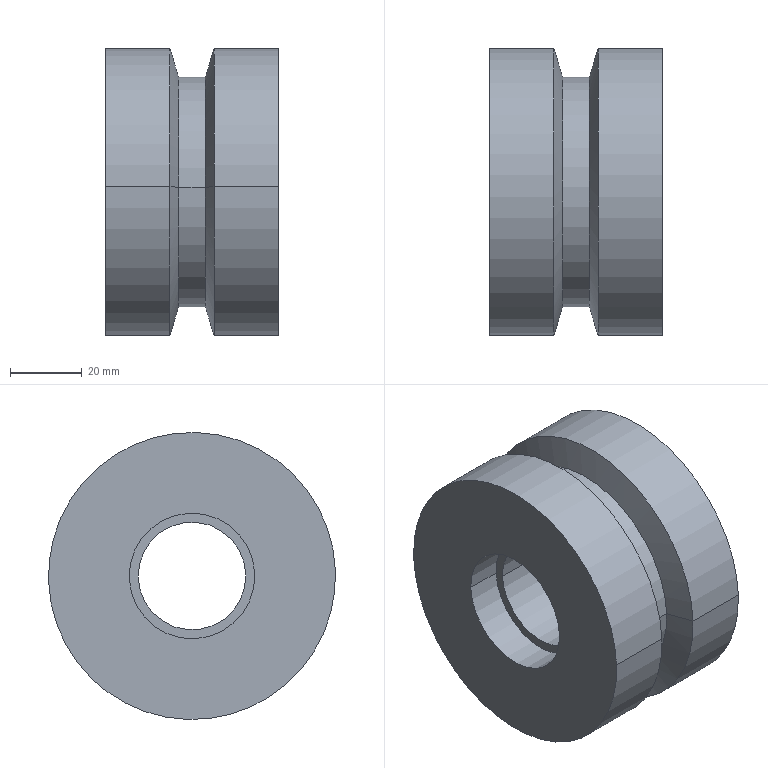Component | SolidWorks | CCD11-00TensioningAssembly-1_CCD05DrivenWheel-1 | 1 solid | 20 faces | box 48 x 80 x 80 mm | volume 184165 mm3 | cylinder 12 | cone 4 | plane 4 | commonest cylinder face diameters 35 x4 80 x4 30 x2 64 x2
build123d program:
from build123d import *


with BuildPart() as part:
    # Sketch1 → Revolve1 (revolve)
    with BuildSketch(Plane.XY, mode=Mode.PRIVATE) as revolve1_sk:
        Polygon((-26.154, 17.5), (-26.154, 40), (-8.304, 40), (-5.904, 32), (1.596, 32), (3.996, 40), (21.846, 40), (21.846, 17.5), (11.846, 17.5), (11.846, 15), (-16.154, 15), (-16.154, 17.5), align=None)
    revolve(revolve1_sk.sketch.rotate(Axis((-155.696, 0, 0), (1, 0, 0)), 90), axis=Axis((-155.696, 0, 0), (1, 0, 0)))


solid = part.part

# Placed as in the assembly
solid = solid.moved(Location((-327.967, 107.251, 149), (0, 0, 0)))
STEP:
#1=COLOUR_RGB('',0.7922,0.8196,0.9333);
#2=FILL_AREA_STYLE_COLOUR('',#1);
#3=FILL_AREA_STYLE('',(#2));
#4=SURFACE_STYLE_FILL_AREA(#3);
#5=SURFACE_SIDE_STYLE('',(#4));
#6=SURFACE_STYLE_USAGE(.BOTH.,#5);
#7=PRESENTATION_STYLE_ASSIGNMENT((#6));
#8=CARTESIAN_POINT('',(-12.446,4.813,5.843));
#9=VERTEX_POINT('',#8);
#10=CARTESIAN_POINT('',(-12.446,3.632,5.889));
#11=VERTEX_POINT('',#10);
#12=CARTESIAN_POINT('',(-12.446,4.222,5.866));
#13=DIRECTION('',(-1.,-0.,0.));
#14=DIRECTION('',(0.,-0.9992,0.03921));
#15=AXIS2_PLACEMENT_3D('',#12,#13,#14);
#16=CIRCLE('',#15,0.5906);
#17=EDGE_CURVE('',#9,#11,#16,.T.);
#18=ORIENTED_EDGE('',*,*,#17,.F.);
#19=CARTESIAN_POINT('',(-13.548,4.813,5.843));
#20=VERTEX_POINT('',#19);
#21=CARTESIAN_POINT('',(-19.042,4.813,5.843));
#22=DIRECTION('',(-1.,-0.,0.));
#23=VECTOR('',#22,39.37);
#24=LINE('',#21,#23);
#25=EDGE_CURVE('',#9,#20,#24,.T.);
#26=ORIENTED_EDGE('',*,*,#25,.T.);
#27=CARTESIAN_POINT('',(-13.548,3.632,5.889));
#28=VERTEX_POINT('',#27);
#29=CARTESIAN_POINT('',(-13.548,4.222,5.866));
#30=DIRECTION('',(-1.,-0.,0.));
#31=DIRECTION('',(0.,-0.9992,0.03921));
#32=AXIS2_PLACEMENT_3D('',#29,#30,#31);
#33=CIRCLE('',#32,0.5906);
#34=EDGE_CURVE('',#20,#28,#33,.T.);
#35=ORIENTED_EDGE('',*,*,#34,.T.);
#36=CARTESIAN_POINT('',(-19.042,3.632,5.889));
#37=DIRECTION('',(-1.,-0.,0.));
#38=VECTOR('',#37,39.37);
#39=LINE('',#36,#38);
#40=EDGE_CURVE('',#11,#28,#39,.T.);
#41=ORIENTED_EDGE('',*,*,#40,.F.);
#42=EDGE_LOOP('',(#18,#26,#35,#41));
#43=FACE_OUTER_BOUND('',#42,.T.);
#44=CARTESIAN_POINT('',(-19.042,4.222,5.866));
#45=DIRECTION('',(-1.,-0.,0.));
#46=DIRECTION('',(0.,-0.9992,0.03921));
#47=AXIS2_PLACEMENT_3D('',#44,#45,#46);
#48=CYLINDRICAL_SURFACE('',#47,0.5906);
#49=ADVANCED_FACE('',(#43),#48,.F.);
#50=CARTESIAN_POINT('',(-12.052,4.911,5.839));
#51=VERTEX_POINT('',#50);
#52=CARTESIAN_POINT('',(-12.052,3.534,5.893));
#53=VERTEX_POINT('',#52);
#54=CARTESIAN_POINT('',(-12.052,4.222,5.866));
#55=DIRECTION('',(-1.,-0.,0.));
#56=DIRECTION('',(0.,-0.9992,0.03921));
#57=AXIS2_PLACEMENT_3D('',#54,#55,#56);
#58=CIRCLE('',#57,0.689);
#59=EDGE_CURVE('',#51,#53,#58,.T.);
#60=ORIENTED_EDGE('',*,*,#59,.F.);
#61=CARTESIAN_POINT('',(-12.446,4.911,5.839));
#62=VERTEX_POINT('',#61);
#63=CARTESIAN_POINT('',(-19.042,4.911,5.839));
#64=DIRECTION('',(-1.,-0.,0.));
#65=VECTOR('',#64,39.37);
#66=LINE('',#63,#65);
#67=EDGE_CURVE('',#51,#62,#66,.T.);
#68=ORIENTED_EDGE('',*,*,#67,.T.);
#69=CARTESIAN_POINT('',(-12.446,3.534,5.893));
#70=VERTEX_POINT('',#69);
#71=CARTESIAN_POINT('',(-12.446,4.222,5.866));
#72=DIRECTION('',(-1.,-0.,0.));
#73=DIRECTION('',(0.,-0.9992,0.03921));
#74=AXIS2_PLACEMENT_3D('',#71,#72,#73);
#75=CIRCLE('',#74,0.689);
#76=EDGE_CURVE('',#62,#70,#75,.T.);
#77=ORIENTED_EDGE('',*,*,#76,.T.);
#78=CARTESIAN_POINT('',(-19.042,3.534,5.893));
#79=DIRECTION('',(-1.,-0.,0.));
#80=VECTOR('',#79,39.37);
#81=LINE('',#78,#80);
#82=EDGE_CURVE('',#53,#70,#81,.T.);
#83=ORIENTED_EDGE('',*,*,#82,.F.);
#84=EDGE_LOOP('',(#60,#68,#77,#83));
#85=FACE_OUTER_BOUND('',#84,.T.);
#86=CARTESIAN_POINT('',(-19.042,4.222,5.866));
#87=DIRECTION('',(-1.,-0.,0.));
#88=DIRECTION('',(0.,-0.9992,0.03921));
#89=AXIS2_PLACEMENT_3D('',#86,#87,#88);
#90=CYLINDRICAL_SURFACE('',#89,0.689);
#91=ADVANCED_FACE('',(#85),#90,.F.);
#92=CARTESIAN_POINT('',(-12.052,2.649,5.928));
#93=VERTEX_POINT('',#92);
#94=CARTESIAN_POINT('',(-12.052,5.796,5.804));
#95=VERTEX_POINT('',#94);
#96=CARTESIAN_POINT('',(-12.052,4.222,5.866));
#97=DIRECTION('',(-1.,-0.,0.));
#98=DIRECTION('',(0.,-0.9992,0.03921));
#99=AXIS2_PLACEMENT_3D('',#96,#97,#98);
#100=CIRCLE('',#99,1.575);
#101=EDGE_CURVE('',#93,#95,#100,.T.);
#102=ORIENTED_EDGE('',*,*,#101,.T.);
#103=CARTESIAN_POINT('',(-12.755,5.796,5.804));
#104=VERTEX_POINT('',#103);
#105=CARTESIAN_POINT('',(-19.042,5.796,5.804));
#106=DIRECTION('',(-1.,-0.,0.));
#107=VECTOR('',#106,39.37);
#108=LINE('',#105,#107);
#109=EDGE_CURVE('',#95,#104,#108,.T.);
#110=ORIENTED_EDGE('',*,*,#109,.T.);
#111=CARTESIAN_POINT('',(-12.755,2.649,5.928));
#112=VERTEX_POINT('',#111);
#113=CARTESIAN_POINT('',(-12.755,4.222,5.866));
#114=DIRECTION('',(-1.,-0.,0.));
#115=DIRECTION('',(0.,-0.9992,0.03921));
#116=AXIS2_PLACEMENT_3D('',#113,#114,#115);
#117=CIRCLE('',#116,1.575);
#118=EDGE_CURVE('',#112,#104,#117,.T.);
#119=ORIENTED_EDGE('',*,*,#118,.F.);
#120=CARTESIAN_POINT('',(-19.042,2.649,5.928));
#121=DIRECTION('',(-1.,-0.,0.));
#122=VECTOR('',#121,39.37);
#123=LINE('',#120,#122);
#124=EDGE_CURVE('',#93,#112,#123,.T.);
#125=ORIENTED_EDGE('',*,*,#124,.F.);
#126=EDGE_LOOP('',(#102,#110,#119,#125));
#127=FACE_OUTER_BOUND('',#126,.T.);
#128=CARTESIAN_POINT('',(-19.042,4.222,5.866));
#129=DIRECTION('',(-1.,-0.,0.));
#130=DIRECTION('',(0.,-0.9992,0.03921));
#131=AXIS2_PLACEMENT_3D('',#128,#129,#130);
#132=CYLINDRICAL_SURFACE('',#131,1.575);
#133=ADVANCED_FACE('',(#127),#132,.T.);
#134=CARTESIAN_POINT('',(-12.849,2.964,5.916));
#135=VERTEX_POINT('',#134);
#136=CARTESIAN_POINT('',(-12.849,5.481,5.817));
#137=VERTEX_POINT('',#136);
#138=CARTESIAN_POINT('',(-12.849,4.222,5.866));
#139=DIRECTION('',(-1.,-0.,0.));
#140=DIRECTION('',(0.,-0.9992,0.03921));
#141=AXIS2_PLACEMENT_3D('',#138,#139,#140);
#142=CIRCLE('',#141,1.26);
#143=EDGE_CURVE('',#135,#137,#142,.T.);
#144=ORIENTED_EDGE('',*,*,#143,.F.);
#145=CARTESIAN_POINT('',(-12.755,2.649,5.928));
#146=DIRECTION('',(0.2873,-0.9571,0.03756));
#147=VECTOR('',#146,39.37);
#148=LINE('',#145,#147);
#149=EDGE_CURVE('',#135,#112,#148,.T.);
#150=ORIENTED_EDGE('',*,*,#149,.T.);
#151=ORIENTED_EDGE('',*,*,#118,.T.);
#152=CARTESIAN_POINT('',(-12.755,5.796,5.804));
#153=DIRECTION('',(0.2873,0.9571,-0.03756));
#154=VECTOR('',#153,39.37);
#155=LINE('',#152,#154);
#156=EDGE_CURVE('',#137,#104,#155,.T.);
#157=ORIENTED_EDGE('',*,*,#156,.F.);
#158=EDGE_LOOP('',(#144,#150,#151,#157));
#159=FACE_OUTER_BOUND('',#158,.T.);
#160=CARTESIAN_POINT('',(-12.755,4.222,5.866));
#161=DIRECTION('',(1.,0.,-0.));
#162=DIRECTION('',(-0.,0.9992,-0.03921));
#163=AXIS2_PLACEMENT_3D('',#160,#161,#162);
#164=CONICAL_SURFACE('',#163,1.575,1.279);
#165=ADVANCED_FACE('',(#159),#164,.T.);
#166=ORIENTED_EDGE('',*,*,#143,.T.);
#167=CARTESIAN_POINT('',(-13.145,5.481,5.817));
#168=VERTEX_POINT('',#167);
#169=CARTESIAN_POINT('',(-19.042,5.481,5.817));
#170=DIRECTION('',(-1.,-0.,0.));
#171=VECTOR('',#170,39.37);
#172=LINE('',#169,#171);
#173=EDGE_CURVE('',#137,#168,#172,.T.);
#174=ORIENTED_EDGE('',*,*,#173,.T.);
#175=CARTESIAN_POINT('',(-13.145,2.964,5.916));
#176=VERTEX_POINT('',#175);
#177=CARTESIAN_POINT('',(-13.145,4.222,5.866));
#178=DIRECTION('',(-1.,-0.,0.));
#179=DIRECTION('',(0.,-0.9992,0.03921));
#180=AXIS2_PLACEMENT_3D('',#177,#178,#179);
#181=CIRCLE('',#180,1.26);
#182=EDGE_CURVE('',#176,#168,#181,.T.);
#183=ORIENTED_EDGE('',*,*,#182,.F.);
#184=CARTESIAN_POINT('',(-19.042,2.964,5.916));
#185=DIRECTION('',(-1.,-0.,0.));
#186=VECTOR('',#185,39.37);
#187=LINE('',#184,#186);
#188=EDGE_CURVE('',#135,#176,#187,.T.);
#189=ORIENTED_EDGE('',*,*,#188,.F.);
#190=EDGE_LOOP('',(#166,#174,#183,#189));
#191=FACE_OUTER_BOUND('',#190,.T.);
#192=CARTESIAN_POINT('',(-19.042,4.222,5.866));
#193=DIRECTION('',(-1.,-0.,0.));
#194=DIRECTION('',(0.,-0.9992,0.03921));
#195=AXIS2_PLACEMENT_3D('',#192,#193,#194);
#196=CYLINDRICAL_SURFACE('',#195,1.26);
#197=ADVANCED_FACE('',(#191),#196,.T.);
#198=ORIENTED_EDGE('',*,*,#182,.T.);
#199=CARTESIAN_POINT('',(-13.239,5.796,5.804));
#200=VERTEX_POINT('',#199);
#201=CARTESIAN_POINT('',(-13.145,5.481,5.817));
#202=DIRECTION('',(-0.2873,0.9571,-0.03756));
#203=VECTOR('',#202,39.37);
#204=LINE('',#201,#203);
#205=EDGE_CURVE('',#168,#200,#204,.T.);
#206=ORIENTED_EDGE('',*,*,#205,.T.);
#207=CARTESIAN_POINT('',(-13.239,2.649,5.928));
#208=VERTEX_POINT('',#207);
#209=CARTESIAN_POINT('',(-13.239,4.222,5.866));
#210=DIRECTION('',(-1.,-0.,0.));
#211=DIRECTION('',(0.,-0.9992,0.03921));
#212=AXIS2_PLACEMENT_3D('',#209,#210,#211);
#213=CIRCLE('',#212,1.575);
#214=EDGE_CURVE('',#208,#200,#213,.T.);
#215=ORIENTED_EDGE('',*,*,#214,.F.);
#216=CARTESIAN_POINT('',(-13.145,2.964,5.916));
#217=DIRECTION('',(-0.2873,-0.9571,0.03756));
#218=VECTOR('',#217,39.37);
#219=LINE('',#216,#218);
#220=EDGE_CURVE('',#176,#208,#219,.T.);
#221=ORIENTED_EDGE('',*,*,#220,.F.);
#222=EDGE_LOOP('',(#198,#206,#215,#221));
#223=FACE_OUTER_BOUND('',#222,.T.);
#224=CARTESIAN_POINT('',(-13.145,4.222,5.866));
#225=DIRECTION('',(-1.,-0.,0.));
#226=DIRECTION('',(0.,-0.9992,0.03921));
#227=AXIS2_PLACEMENT_3D('',#224,#225,#226);
#228=CONICAL_SURFACE('',#227,1.26,1.279);
#229=ADVANCED_FACE('',(#223),#228,.T.);
#230=ORIENTED_EDGE('',*,*,#214,.T.);
#231=CARTESIAN_POINT('',(-13.942,5.796,5.804));
#232=VERTEX_POINT('',#231);
#233=CARTESIAN_POINT('',(-19.042,5.796,5.804));
#234=DIRECTION('',(-1.,-0.,0.));
#235=VECTOR('',#234,39.37);
#236=LINE('',#233,#235);
#237=EDGE_CURVE('',#200,#232,#236,.T.);
#238=ORIENTED_EDGE('',*,*,#237,.T.);
#239=CARTESIAN_POINT('',(-13.942,2.649,5.928));
#240=VERTEX_POINT('',#239);
#241=CARTESIAN_POINT('',(-13.942,4.222,5.866));
#242=DIRECTION('',(-1.,-0.,0.));
#243=DIRECTION('',(0.,-0.9992,0.03921));
#244=AXIS2_PLACEMENT_3D('',#241,#242,#243);
#245=CIRCLE('',#244,1.575);
#246=EDGE_CURVE('',#240,#232,#245,.T.);
#247=ORIENTED_EDGE('',*,*,#246,.F.);
#248=CARTESIAN_POINT('',(-19.042,2.649,5.928));
#249=DIRECTION('',(-1.,-0.,0.));
#250=VECTOR('',#249,39.37);
#251=LINE('',#248,#250);
#252=EDGE_CURVE('',#208,#240,#251,.T.);
#253=ORIENTED_EDGE('',*,*,#252,.F.);
#254=EDGE_LOOP('',(#230,#238,#247,#253));
#255=FACE_OUTER_BOUND('',#254,.T.);
#256=CARTESIAN_POINT('',(-19.042,4.222,5.866));
#257=DIRECTION('',(-1.,-0.,0.));
#258=DIRECTION('',(0.,-0.9992,0.03921));
#259=AXIS2_PLACEMENT_3D('',#256,#257,#258);
#260=CYLINDRICAL_SURFACE('',#259,1.575);
#261=ADVANCED_FACE('',(#255),#260,.T.);
#262=CARTESIAN_POINT('',(-13.548,4.911,5.839));
#263=VERTEX_POINT('',#262);
#264=CARTESIAN_POINT('',(-13.548,3.534,5.893));
#265=VERTEX_POINT('',#264);
#266=CARTESIAN_POINT('',(-13.548,4.222,5.866));
#267=DIRECTION('',(-1.,-0.,0.));
#268=DIRECTION('',(0.,-0.9992,0.03921));
#269=AXIS2_PLACEMENT_3D('',#266,#267,#268);
#270=CIRCLE('',#269,0.689);
#271=EDGE_CURVE('',#263,#265,#270,.T.);
#272=ORIENTED_EDGE('',*,*,#271,.F.);
#273=CARTESIAN_POINT('',(-13.942,4.911,5.839));
#274=VERTEX_POINT('',#273);
#275=CARTESIAN_POINT('',(-19.042,4.911,5.839));
#276=DIRECTION('',(-1.,-0.,0.));
#277=VECTOR('',#276,39.37);
#278=LINE('',#275,#277);
#279=EDGE_CURVE('',#263,#274,#278,.T.);
#280=ORIENTED_EDGE('',*,*,#279,.T.);
#281=CARTESIAN_POINT('',(-13.942,3.534,5.893));
#282=VERTEX_POINT('',#281);
#283=CARTESIAN_POINT('',(-13.942,4.222,5.866));
#284=DIRECTION('',(-1.,-0.,0.));
#285=DIRECTION('',(0.,-0.9992,0.03921));
#286=AXIS2_PLACEMENT_3D('',#283,#284,#285);
#287=CIRCLE('',#286,0.689);
#288=EDGE_CURVE('',#274,#282,#287,.T.);
#289=ORIENTED_EDGE('',*,*,#288,.T.);
#290=CARTESIAN_POINT('',(-19.042,3.534,5.893));
#291=DIRECTION('',(-1.,-0.,0.));
#292=VECTOR('',#291,39.37);
#293=LINE('',#290,#292);
#294=EDGE_CURVE('',#265,#282,#293,.T.);
#295=ORIENTED_EDGE('',*,*,#294,.F.);
#296=EDGE_LOOP('',(#272,#280,#289,#295));
#297=FACE_OUTER_BOUND('',#296,.T.);
#298=CARTESIAN_POINT('',(-19.042,4.222,5.866));
#299=DIRECTION('',(-1.,-0.,0.));
#300=DIRECTION('',(0.,-0.9992,0.03921));
#301=AXIS2_PLACEMENT_3D('',#298,#299,#300);
#302=CYLINDRICAL_SURFACE('',#301,0.689);
#303=ADVANCED_FACE('',(#297),#302,.F.);
#304=ORIENTED_EDGE('',*,*,#279,.F.);
#305=CARTESIAN_POINT('',(-13.548,4.222,5.866));
#306=DIRECTION('',(-1.,-0.,0.));
#307=DIRECTION('',(0.,-0.9992,0.03921));
#308=AXIS2_PLACEMENT_3D('',#305,#306,#307);
#309=CIRCLE('',#308,0.689);
#310=EDGE_CURVE('',#265,#263,#309,.T.);
#311=ORIENTED_EDGE('',*,*,#310,.F.);
#312=ORIENTED_EDGE('',*,*,#294,.T.);
#313=CARTESIAN_POINT('',(-13.942,4.222,5.866));
#314=DIRECTION('',(-1.,-0.,0.));
#315=DIRECTION('',(0.,-0.9992,0.03921));
#316=AXIS2_PLACEMENT_3D('',#313,#314,#315);
#317=CIRCLE('',#316,0.689);
#318=EDGE_CURVE('',#282,#274,#317,.T.);
#319=ORIENTED_EDGE('',*,*,#318,.T.);
#320=EDGE_LOOP('',(#304,#311,#312,#319));
#321=FACE_OUTER_BOUND('',#320,.T.);
#322=CARTESIAN_POINT('',(-19.042,4.222,5.866));
#323=DIRECTION('',(-1.,-0.,0.));
#324=DIRECTION('',(0.,-0.9992,0.03921));
#325=AXIS2_PLACEMENT_3D('',#322,#323,#324);
#326=CYLINDRICAL_SURFACE('',#325,0.689);
#327=ADVANCED_FACE('',(#321),#326,.F.);
#328=ORIENTED_EDGE('',*,*,#318,.F.);
#329=ORIENTED_EDGE('',*,*,#288,.F.);
#330=EDGE_LOOP('',(#328,#329));
#331=FACE_BOUND('',#330,.T.);
#332=ORIENTED_EDGE('',*,*,#246,.T.);
#333=CARTESIAN_POINT('',(-13.942,4.222,5.866));
#334=DIRECTION('',(-1.,-0.,0.));
#335=DIRECTION('',(0.,-0.9992,0.03921));
#336=AXIS2_PLACEMENT_3D('',#333,#334,#335);
#337=CIRCLE('',#336,1.575);
#338=EDGE_CURVE('',#232,#240,#337,.T.);
#339=ORIENTED_EDGE('',*,*,#338,.T.);
#340=EDGE_LOOP('',(#332,#339));
#341=FACE_OUTER_BOUND('',#340,.T.);
#342=CARTESIAN_POINT('',(-13.942,4.25,6.555));
#343=DIRECTION('',(1.,0.,-0.));
#344=DIRECTION('',(-0.,0.9992,-0.03921));
#345=AXIS2_PLACEMENT_3D('',#342,#343,#344);
#346=PLANE('',#345);
#347=ADVANCED_FACE('',(#331,#341),#346,.F.);
#348=ORIENTED_EDGE('',*,*,#237,.F.);
#349=CARTESIAN_POINT('',(-13.239,4.222,5.866));
#350=DIRECTION('',(-1.,-0.,0.));
#351=DIRECTION('',(0.,-0.9992,0.03921));
#352=AXIS2_PLACEMENT_3D('',#349,#350,#351);
#353=CIRCLE('',#352,1.575);
#354=EDGE_CURVE('',#200,#208,#353,.T.);
#355=ORIENTED_EDGE('',*,*,#354,.T.);
#356=ORIENTED_EDGE('',*,*,#252,.T.);
#357=ORIENTED_EDGE('',*,*,#338,.F.);
#358=EDGE_LOOP('',(#348,#355,#356,#357));
#359=FACE_OUTER_BOUND('',#358,.T.);
#360=CARTESIAN_POINT('',(-19.042,4.222,5.866));
#361=DIRECTION('',(-1.,-0.,0.));
#362=DIRECTION('',(0.,-0.9992,0.03921));
#363=AXIS2_PLACEMENT_3D('',#360,#361,#362);
#364=CYLINDRICAL_SURFACE('',#363,1.575);
#365=ADVANCED_FACE('',(#359),#364,.T.);
#366=ORIENTED_EDGE('',*,*,#205,.F.);
#367=CARTESIAN_POINT('',(-13.145,4.222,5.866));
#368=DIRECTION('',(-1.,-0.,0.));
#369=DIRECTION('',(0.,-0.9992,0.03921));
#370=AXIS2_PLACEMENT_3D('',#367,#368,#369);
#371=CIRCLE('',#370,1.26);
#372=EDGE_CURVE('',#168,#176,#371,.T.);
#373=ORIENTED_EDGE('',*,*,#372,.T.);
#374=ORIENTED_EDGE('',*,*,#220,.T.);
#375=ORIENTED_EDGE('',*,*,#354,.F.);
#376=EDGE_LOOP('',(#366,#373,#374,#375));
#377=FACE_OUTER_BOUND('',#376,.T.);
#378=CARTESIAN_POINT('',(-13.145,4.222,5.866));
#379=DIRECTION('',(-1.,-0.,0.));
#380=DIRECTION('',(0.,-0.9992,0.03921));
#381=AXIS2_PLACEMENT_3D('',#378,#379,#380);
#382=CONICAL_SURFACE('',#381,1.26,1.279);
#383=ADVANCED_FACE('',(#377),#382,.T.);
#384=ORIENTED_EDGE('',*,*,#173,.F.);
#385=CARTESIAN_POINT('',(-12.849,4.222,5.866));
#386=DIRECTION('',(-1.,-0.,0.));
#387=DIRECTION('',(0.,-0.9992,0.03921));
#388=AXIS2_PLACEMENT_3D('',#385,#386,#387);
#389=CIRCLE('',#388,1.26);
#390=EDGE_CURVE('',#137,#135,#389,.T.);
#391=ORIENTED_EDGE('',*,*,#390,.T.);
#392=ORIENTED_EDGE('',*,*,#188,.T.);
#393=ORIENTED_EDGE('',*,*,#372,.F.);
#394=EDGE_LOOP('',(#384,#391,#392,#393));
#395=FACE_OUTER_BOUND('',#394,.T.);
#396=CARTESIAN_POINT('',(-19.042,4.222,5.866));
#397=DIRECTION('',(-1.,-0.,0.));
#398=DIRECTION('',(0.,-0.9992,0.03921));
#399=AXIS2_PLACEMENT_3D('',#396,#397,#398);
#400=CYLINDRICAL_SURFACE('',#399,1.26);
#401=ADVANCED_FACE('',(#395),#400,.T.);
#402=ORIENTED_EDGE('',*,*,#149,.F.);
#403=ORIENTED_EDGE('',*,*,#390,.F.);
#404=ORIENTED_EDGE('',*,*,#156,.T.);
#405=CARTESIAN_POINT('',(-12.755,4.222,5.866));
#406=DIRECTION('',(-1.,-0.,0.));
#407=DIRECTION('',(0.,-0.9992,0.03921));
#408=AXIS2_PLACEMENT_3D('',#405,#406,#407);
#409=CIRCLE('',#408,1.575);
#410=EDGE_CURVE('',#104,#112,#409,.T.);
#411=ORIENTED_EDGE('',*,*,#410,.T.);
#412=EDGE_LOOP('',(#402,#403,#404,#411));
#413=FACE_OUTER_BOUND('',#412,.T.);
#414=CARTESIAN_POINT('',(-12.755,4.222,5.866));
#415=DIRECTION('',(1.,0.,-0.));
#416=DIRECTION('',(-0.,0.9992,-0.03921));
#417=AXIS2_PLACEMENT_3D('',#414,#415,#416);
#418=CONICAL_SURFACE('',#417,1.575,1.279);
#419=ADVANCED_FACE('',(#413),#418,.T.);
#420=ORIENTED_EDGE('',*,*,#109,.F.);
#421=CARTESIAN_POINT('',(-12.052,4.222,5.866));
#422=DIRECTION('',(-1.,-0.,0.));
#423=DIRECTION('',(0.,-0.9992,0.03921));
#424=AXIS2_PLACEMENT_3D('',#421,#422,#423);
#425=CIRCLE('',#424,1.575);
#426=EDGE_CURVE('',#95,#93,#425,.T.);
#427=ORIENTED_EDGE('',*,*,#426,.T.);
#428=ORIENTED_EDGE('',*,*,#124,.T.);
#429=ORIENTED_EDGE('',*,*,#410,.F.);
#430=EDGE_LOOP('',(#420,#427,#428,#429));
#431=FACE_OUTER_BOUND('',#430,.T.);
#432=CARTESIAN_POINT('',(-19.042,4.222,5.866));
#433=DIRECTION('',(-1.,-0.,0.));
#434=DIRECTION('',(0.,-0.9992,0.03921));
#435=AXIS2_PLACEMENT_3D('',#432,#433,#434);
#436=CYLINDRICAL_SURFACE('',#435,1.575);
#437=ADVANCED_FACE('',(#431),#436,.T.);
#438=ORIENTED_EDGE('',*,*,#101,.F.);
#439=ORIENTED_EDGE('',*,*,#426,.F.);
#440=EDGE_LOOP('',(#438,#439));
#441=FACE_OUTER_BOUND('',#440,.T.);
#442=CARTESIAN_POINT('',(-12.052,4.222,5.866));
#443=DIRECTION('',(-1.,-0.,0.));
#444=DIRECTION('',(0.,-0.9992,0.03921));
#445=AXIS2_PLACEMENT_3D('',#442,#443,#444);
#446=CIRCLE('',#445,0.689);
#447=EDGE_CURVE('',#53,#51,#446,.T.);
#448=ORIENTED_EDGE('',*,*,#447,.T.);
#449=ORIENTED_EDGE('',*,*,#59,.T.);
#450=EDGE_LOOP('',(#448,#449));
#451=FACE_BOUND('',#450,.T.);
#452=CARTESIAN_POINT('',(-12.052,4.284,7.44));
#453=DIRECTION('',(-1.,-0.,0.));
#454=DIRECTION('',(0.,-0.9992,0.03921));
#455=AXIS2_PLACEMENT_3D('',#452,#453,#454);
#456=PLANE('',#455);
#457=ADVANCED_FACE('',(#441,#451),#456,.F.);
#458=ORIENTED_EDGE('',*,*,#67,.F.);
#459=ORIENTED_EDGE('',*,*,#447,.F.);
#460=ORIENTED_EDGE('',*,*,#82,.T.);
#461=CARTESIAN_POINT('',(-12.446,4.222,5.866));
#462=DIRECTION('',(-1.,-0.,0.));
#463=DIRECTION('',(0.,-0.9992,0.03921));
#464=AXIS2_PLACEMENT_3D('',#461,#462,#463);
#465=CIRCLE('',#464,0.689);
#466=EDGE_CURVE('',#70,#62,#465,.T.);
#467=ORIENTED_EDGE('',*,*,#466,.T.);
#468=EDGE_LOOP('',(#458,#459,#460,#467));
#469=FACE_OUTER_BOUND('',#468,.T.);
#470=CARTESIAN_POINT('',(-19.042,4.222,5.866));
#471=DIRECTION('',(-1.,-0.,0.));
#472=DIRECTION('',(0.,-0.9992,0.03921));
#473=AXIS2_PLACEMENT_3D('',#470,#471,#472);
#474=CYLINDRICAL_SURFACE('',#473,0.689);
#475=ADVANCED_FACE('',(#469),#474,.F.);
#476=ORIENTED_EDGE('',*,*,#466,.F.);
#477=ORIENTED_EDGE('',*,*,#76,.F.);
#478=EDGE_LOOP('',(#476,#477));
#479=FACE_OUTER_BOUND('',#478,.T.);
#480=CARTESIAN_POINT('',(-12.446,4.222,5.866));
#481=DIRECTION('',(-1.,-0.,0.));
#482=DIRECTION('',(0.,-0.9992,0.03921));
#483=AXIS2_PLACEMENT_3D('',#480,#481,#482);
#484=CIRCLE('',#483,0.5906);
#485=EDGE_CURVE('',#11,#9,#484,.T.);
#486=ORIENTED_EDGE('',*,*,#485,.T.);
#487=ORIENTED_EDGE('',*,*,#17,.T.);
#488=EDGE_LOOP('',(#486,#487));
#489=FACE_BOUND('',#488,.T.);
#490=CARTESIAN_POINT('',(-12.446,4.25,6.555));
#491=DIRECTION('',(-1.,-0.,0.));
#492=DIRECTION('',(0.,-0.9992,0.03921));
#493=AXIS2_PLACEMENT_3D('',#490,#491,#492);
#494=PLANE('',#493);
#495=ADVANCED_FACE('',(#479,#489),#494,.F.);
#496=ORIENTED_EDGE('',*,*,#25,.F.);
#497=ORIENTED_EDGE('',*,*,#485,.F.);
#498=ORIENTED_EDGE('',*,*,#40,.T.);
#499=CARTESIAN_POINT('',(-13.548,4.222,5.866));
#500=DIRECTION('',(-1.,-0.,0.));
#501=DIRECTION('',(0.,-0.9992,0.03921));
#502=AXIS2_PLACEMENT_3D('',#499,#500,#501);
#503=CIRCLE('',#502,0.5906);
#504=EDGE_CURVE('',#28,#20,#503,.T.);
#505=ORIENTED_EDGE('',*,*,#504,.T.);
#506=EDGE_LOOP('',(#496,#497,#498,#505));
#507=FACE_OUTER_BOUND('',#506,.T.);
#508=CARTESIAN_POINT('',(-19.042,4.222,5.866));
#509=DIRECTION('',(-1.,-0.,0.));
#510=DIRECTION('',(0.,-0.9992,0.03921));
#511=AXIS2_PLACEMENT_3D('',#508,#509,#510);
#512=CYLINDRICAL_SURFACE('',#511,0.5906);
#513=ADVANCED_FACE('',(#507),#512,.F.);
#514=ORIENTED_EDGE('',*,*,#504,.F.);
#515=ORIENTED_EDGE('',*,*,#34,.F.);
#516=EDGE_LOOP('',(#514,#515));
#517=FACE_BOUND('',#516,.T.);
#518=ORIENTED_EDGE('',*,*,#310,.T.);
#519=ORIENTED_EDGE('',*,*,#271,.T.);
#520=EDGE_LOOP('',(#518,#519));
#521=FACE_OUTER_BOUND('',#520,.T.);
#522=CARTESIAN_POINT('',(-13.548,4.246,6.456));
#523=DIRECTION('',(1.,0.,-0.));
#524=DIRECTION('',(-0.,0.9992,-0.03921));
#525=AXIS2_PLACEMENT_3D('',#522,#523,#524);
#526=PLANE('',#525);
#527=ADVANCED_FACE('',(#517,#521),#526,.F.);
#528=CLOSED_SHELL('',(#49,#91,#133,#165,#197,#229,#261,#303,#327,#347,#365,#383,#401,#419,#437,#457,#475,#495,#513,#527));
#529=MANIFOLD_SOLID_BREP('',#528);
#530=STYLED_ITEM('',(#7),#529);
#531=PRESENTATION_LAYER_ASSIGNMENT('','',(#530));
#532=CARTESIAN_POINT('',(0.,0.,0.));
#533=DIRECTION('',(0.,0.,1.));
#534=DIRECTION('',(1.,0.,0.));
#535=AXIS2_PLACEMENT_3D('',#532,#533,#534);
#536=(LENGTH_UNIT()NAMED_UNIT(*)SI_UNIT($,.METRE.));
#537=LENGTH_MEASURE_WITH_UNIT(LENGTH_MEASURE(0.0254),#536);
#538=DIMENSIONAL_EXPONENTS(1.,0.,0.,0.,0.,0.,0.);
#539=(CONVERSION_BASED_UNIT('',#537)LENGTH_UNIT()NAMED_UNIT(#538));
#540=UNCERTAINTY_MEASURE_WITH_UNIT(LENGTH_MEASURE(0.00001),#539,'','');
#541=(NAMED_UNIT(*)PLANE_ANGLE_UNIT()SI_UNIT($,.RADIAN.));
#542=(NAMED_UNIT(*)SI_UNIT($,.STERADIAN.)SOLID_ANGLE_UNIT());
#543=(GEOMETRIC_REPRESENTATION_CONTEXT(3)GLOBAL_UNCERTAINTY_ASSIGNED_CONTEXT((#540))GLOBAL_UNIT_ASSIGNED_CONTEXT((#539,#541,#542))REPRESENTATION_CONTEXT('',''));
#544=ADVANCED_BREP_SHAPE_REPRESENTATION('',(#529,#535),#543);
#545=(LENGTH_UNIT()NAMED_UNIT(*)SI_UNIT($,.METRE.));
#546=LENGTH_MEASURE_WITH_UNIT(LENGTH_MEASURE(0.0254),#545);
#547=DIMENSIONAL_EXPONENTS(1.,0.,0.,0.,0.,0.,0.);
#548=(CONVERSION_BASED_UNIT('',#546)LENGTH_UNIT()NAMED_UNIT(#547));
#549=UNCERTAINTY_MEASURE_WITH_UNIT(LENGTH_MEASURE(0.00001),#548,'','');
#550=(NAMED_UNIT(*)PLANE_ANGLE_UNIT()SI_UNIT($,.RADIAN.));
#551=(NAMED_UNIT(*)SI_UNIT($,.STERADIAN.)SOLID_ANGLE_UNIT());
#552=(GEOMETRIC_REPRESENTATION_CONTEXT(3)GLOBAL_UNCERTAINTY_ASSIGNED_CONTEXT((#549))GLOBAL_UNIT_ASSIGNED_CONTEXT((#548,#550,#551))REPRESENTATION_CONTEXT('',''));
#553=MECHANICAL_DESIGN_GEOMETRIC_PRESENTATION_REPRESENTATION('',(#530),#552);